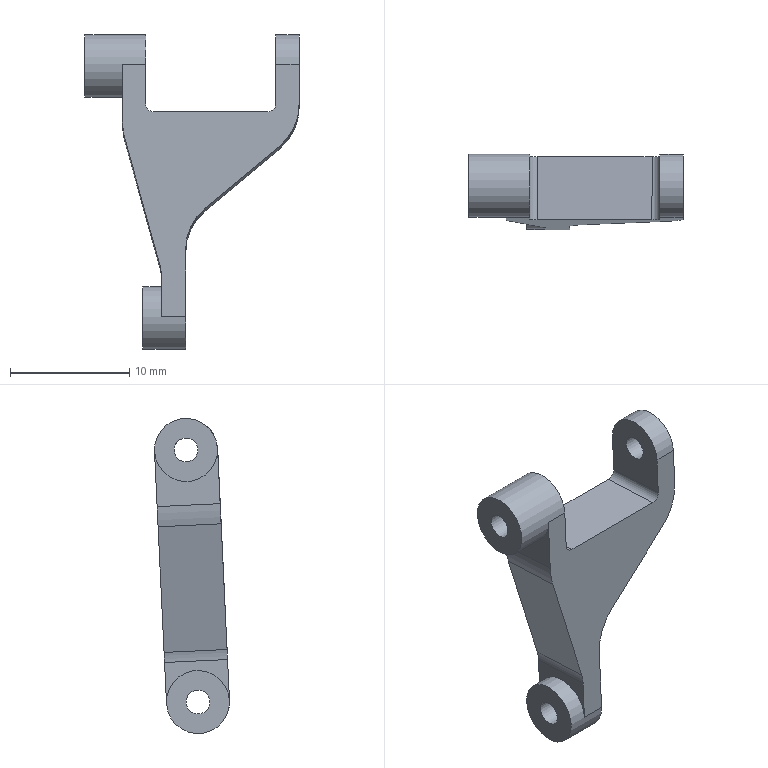Component | NX | ROTATING_ROD_2 | 1 solid | 25 faces | volume 808 mm3 | plane 13 | cylinder 12 | commonest cylinder face diameters 5.292 x3 2 x3 1.323 x2 9.144 x2 6.35 x1 12.7 x1